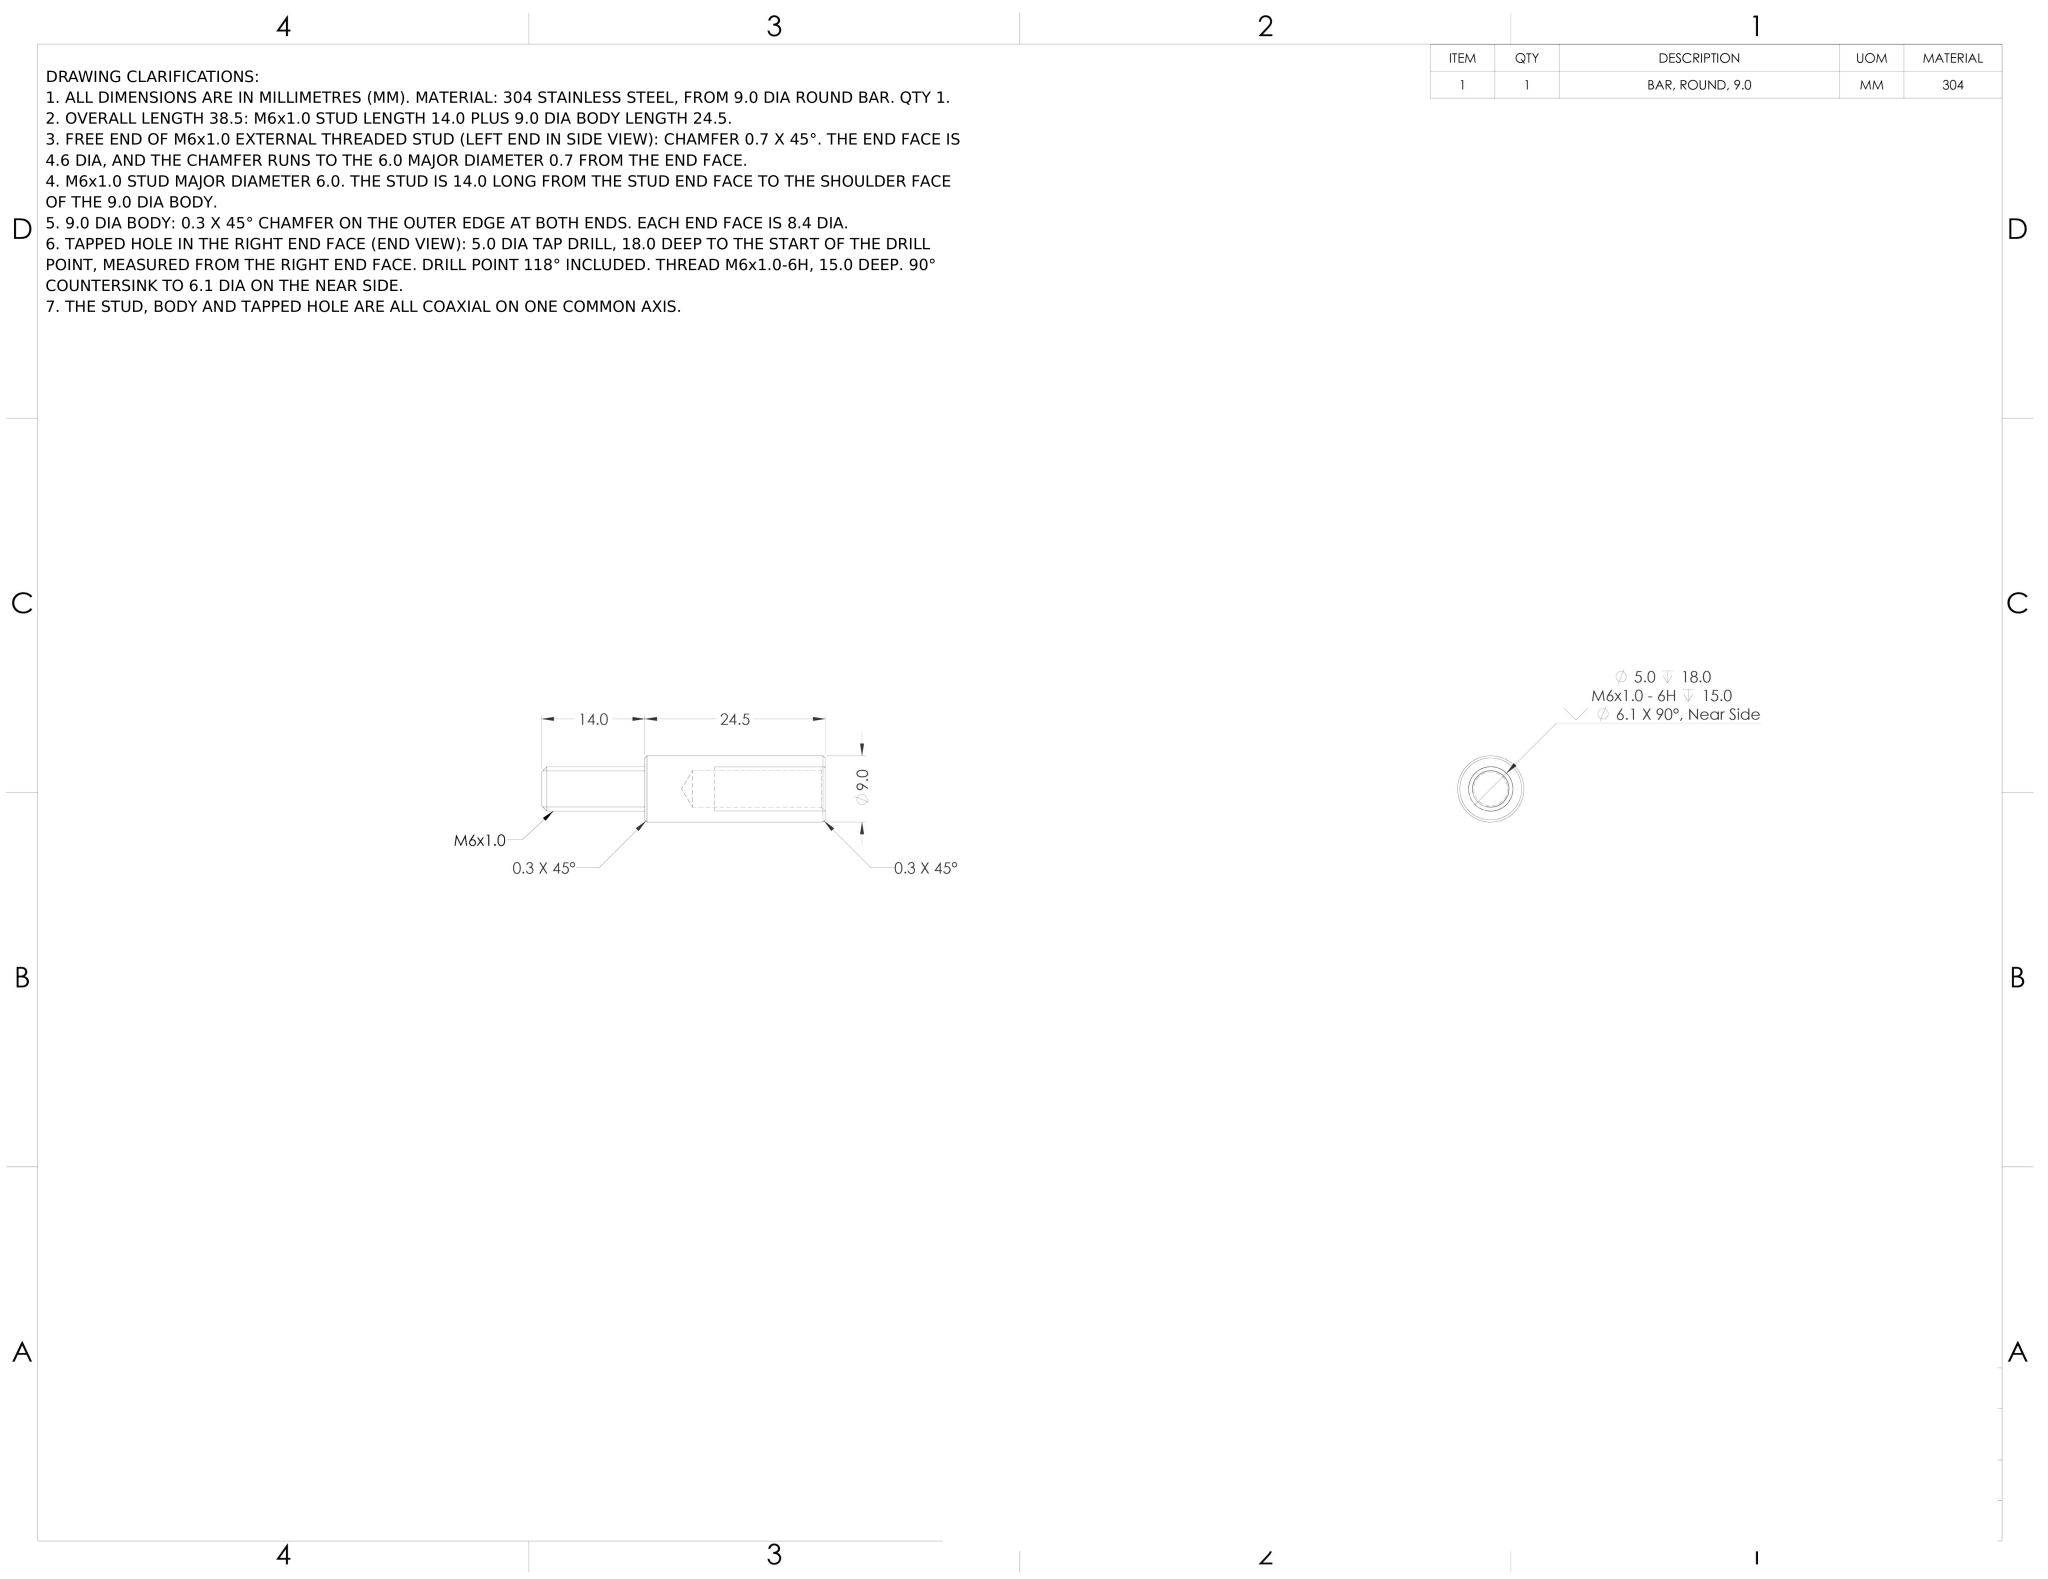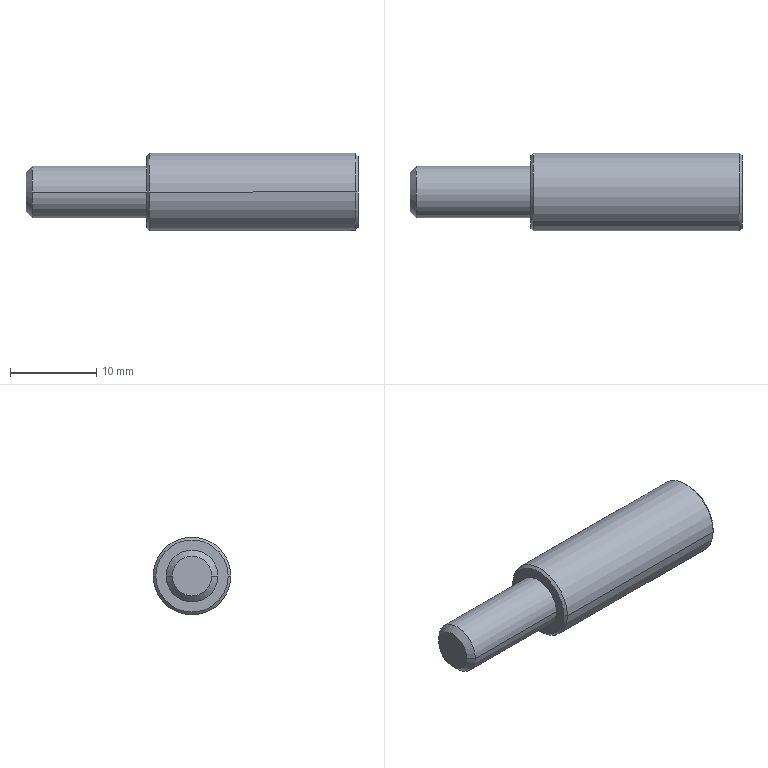Part | NX | mm | Stepped Hollow Cylindrical Connector | 1 solid | 19 faces | box 38.5 x 9 x 9 mm | volume 1582 mm3 | cone 10 | cylinder 6 | plane 3 | commonest cylinder face diameters 5 x2 6 x2 9 x2
STEP:
#1=COLOUR_RGB('',0.9098,0.9176,0.949);
#2=FILL_AREA_STYLE_COLOUR('',#1);
#3=FILL_AREA_STYLE('',(#2));
#4=SURFACE_STYLE_FILL_AREA(#3);
#5=SURFACE_SIDE_STYLE('',(#4));
#6=SURFACE_STYLE_USAGE(.BOTH.,#5);
#7=PRESENTATION_STYLE_ASSIGNMENT((#6));
#8=CARTESIAN_POINT('',(-5.75,0.,2.5));
#9=VERTEX_POINT('',#8);
#10=CARTESIAN_POINT('',(11.725,0.,2.5));
#11=VERTEX_POINT('',#10);
#12=CARTESIAN_POINT('',(12.25,0.,2.5));
#13=DIRECTION('',(1.,0.,0.));
#14=VECTOR('',#13,1000.);
#15=LINE('',#12,#14);
#16=EDGE_CURVE('',#9,#11,#15,.T.);
#17=ORIENTED_EDGE('',*,*,#16,.F.);
#18=CARTESIAN_POINT('',(-5.75,0.,-2.5));
#19=VERTEX_POINT('',#18);
#20=CARTESIAN_POINT('',(-5.75,0.,-0.));
#21=DIRECTION('',(1.,0.,0.));
#22=DIRECTION('',(0.,0.,-1.));
#23=AXIS2_PLACEMENT_3D('',#20,#21,#22);
#24=CIRCLE('',#23,2.5);
#25=EDGE_CURVE('',#19,#9,#24,.T.);
#26=ORIENTED_EDGE('',*,*,#25,.F.);
#27=CARTESIAN_POINT('',(11.725,0.,-2.5));
#28=VERTEX_POINT('',#27);
#29=CARTESIAN_POINT('',(12.25,0.,-2.5));
#30=DIRECTION('',(1.,0.,0.));
#31=VECTOR('',#30,1000.);
#32=LINE('',#29,#31);
#33=EDGE_CURVE('',#19,#28,#32,.T.);
#34=ORIENTED_EDGE('',*,*,#33,.T.);
#35=CARTESIAN_POINT('',(11.725,0.,0.));
#36=DIRECTION('',(1.,0.,0.));
#37=DIRECTION('',(0.,0.,-1.));
#38=AXIS2_PLACEMENT_3D('',#35,#36,#37);
#39=CIRCLE('',#38,2.5);
#40=EDGE_CURVE('',#28,#11,#39,.T.);
#41=ORIENTED_EDGE('',*,*,#40,.T.);
#42=EDGE_LOOP('',(#17,#26,#34,#41));
#43=FACE_OUTER_BOUND('',#42,.T.);
#44=CARTESIAN_POINT('',(12.25,0.,0.));
#45=DIRECTION('',(1.,0.,0.));
#46=DIRECTION('',(0.,0.,-1.));
#47=AXIS2_PLACEMENT_3D('',#44,#45,#46);
#48=CYLINDRICAL_SURFACE('',#47,2.5);
#49=ADVANCED_FACE('',(#43),#48,.F.);
#50=STYLED_ITEM('',(#7),#49);
#51=PRESENTATION_LAYER_ASSIGNMENT('','',(#50));
#52=COLOUR_RGB('',0.9098,0.9176,0.949);
#53=FILL_AREA_STYLE_COLOUR('',#52);
#54=FILL_AREA_STYLE('',(#53));
#55=SURFACE_STYLE_FILL_AREA(#54);
#56=SURFACE_SIDE_STYLE('',(#55));
#57=SURFACE_STYLE_USAGE(.BOTH.,#56);
#58=PRESENTATION_STYLE_ASSIGNMENT((#57));
#59=CARTESIAN_POINT('',(-12.25,3.,-0.));
#60=VERTEX_POINT('',#59);
#61=CARTESIAN_POINT('',(-25.55,3.,-0.));
#62=VERTEX_POINT('',#61);
#63=CARTESIAN_POINT('',(-34.59,3.,-0.));
#64=DIRECTION('',(-1.,-0.,0.));
#65=VECTOR('',#64,1000.);
#66=LINE('',#63,#65);
#67=EDGE_CURVE('',#60,#62,#66,.T.);
#68=ORIENTED_EDGE('',*,*,#67,.F.);
#69=CARTESIAN_POINT('',(-12.25,-3.,-0.));
#70=VERTEX_POINT('',#69);
#71=CARTESIAN_POINT('',(-12.25,0.,-0.));
#72=DIRECTION('',(-1.,-0.,0.));
#73=DIRECTION('',(0.,-1.,0.));
#74=AXIS2_PLACEMENT_3D('',#71,#72,#73);
#75=CIRCLE('',#74,3.);
#76=EDGE_CURVE('',#60,#70,#75,.T.);
#77=ORIENTED_EDGE('',*,*,#76,.T.);
#78=CARTESIAN_POINT('',(-25.55,-3.,-0.));
#79=VERTEX_POINT('',#78);
#80=CARTESIAN_POINT('',(-34.59,-3.,-0.));
#81=DIRECTION('',(-1.,-0.,0.));
#82=VECTOR('',#81,1000.);
#83=LINE('',#80,#82);
#84=EDGE_CURVE('',#70,#79,#83,.T.);
#85=ORIENTED_EDGE('',*,*,#84,.T.);
#86=CARTESIAN_POINT('',(-25.55,0.,-0.));
#87=DIRECTION('',(1.,0.,0.));
#88=DIRECTION('',(0.,1.,0.));
#89=AXIS2_PLACEMENT_3D('',#86,#87,#88);
#90=CIRCLE('',#89,3.);
#91=EDGE_CURVE('',#79,#62,#90,.T.);
#92=ORIENTED_EDGE('',*,*,#91,.T.);
#93=EDGE_LOOP('',(#68,#77,#85,#92));
#94=FACE_OUTER_BOUND('',#93,.T.);
#95=CARTESIAN_POINT('',(-34.59,0.,-0.));
#96=DIRECTION('',(-1.,-0.,0.));
#97=DIRECTION('',(0.,-1.,0.));
#98=AXIS2_PLACEMENT_3D('',#95,#96,#97);
#99=CYLINDRICAL_SURFACE('',#98,3.);
#100=ADVANCED_FACE('',(#94),#99,.T.);
#101=STYLED_ITEM('',(#58),#100);
#102=(LENGTH_UNIT()NAMED_UNIT(*)SI_UNIT(.MILLI.,.METRE.));
#103=UNCERTAINTY_MEASURE_WITH_UNIT(LENGTH_MEASURE(0.00001),#102,'','');
#104=(NAMED_UNIT(*)PLANE_ANGLE_UNIT()SI_UNIT($,.RADIAN.));
#105=(NAMED_UNIT(*)SI_UNIT($,.STERADIAN.)SOLID_ANGLE_UNIT());
#106=(GEOMETRIC_REPRESENTATION_CONTEXT(3)GLOBAL_UNCERTAINTY_ASSIGNED_CONTEXT((#103))GLOBAL_UNIT_ASSIGNED_CONTEXT((#102,#104,#105))REPRESENTATION_CONTEXT('',''));
#107=MECHANICAL_DESIGN_GEOMETRIC_PRESENTATION_REPRESENTATION('',(#101),#106);
#108=COLOUR_RGB('',0.9098,0.9176,0.949);
#109=FILL_AREA_STYLE_COLOUR('',#108);
#110=FILL_AREA_STYLE('',(#109));
#111=SURFACE_STYLE_FILL_AREA(#110);
#112=SURFACE_SIDE_STYLE('',(#111));
#113=SURFACE_STYLE_USAGE(.BOTH.,#112);
#114=PRESENTATION_STYLE_ASSIGNMENT((#113));
#115=CARTESIAN_POINT('',(-12.25,-4.2,-0.));
#116=VERTEX_POINT('',#115);
#117=CARTESIAN_POINT('',(-12.25,4.2,-0.));
#118=VERTEX_POINT('',#117);
#119=CARTESIAN_POINT('',(-12.25,0.,-0.));
#120=DIRECTION('',(-1.,-0.,0.));
#121=DIRECTION('',(0.,1.,0.));
#122=AXIS2_PLACEMENT_3D('',#119,#120,#121);
#123=CIRCLE('',#122,4.2);
#124=EDGE_CURVE('',#116,#118,#123,.T.);
#125=ORIENTED_EDGE('',*,*,#124,.F.);
#126=CARTESIAN_POINT('',(-11.95,-4.5,-0.));
#127=VERTEX_POINT('',#126);
#128=CARTESIAN_POINT('',(-12.25,-4.2,-0.));
#129=DIRECTION('',(0.7071,-0.7071,0.));
#130=VECTOR('',#129,1000.);
#131=LINE('',#128,#130);
#132=EDGE_CURVE('',#116,#127,#131,.T.);
#133=ORIENTED_EDGE('',*,*,#132,.T.);
#134=CARTESIAN_POINT('',(-11.95,4.5,-0.));
#135=VERTEX_POINT('',#134);
#136=CARTESIAN_POINT('',(-11.95,0.,-0.));
#137=DIRECTION('',(1.,0.,0.));
#138=DIRECTION('',(0.,1.,0.));
#139=AXIS2_PLACEMENT_3D('',#136,#137,#138);
#140=CIRCLE('',#139,4.5);
#141=EDGE_CURVE('',#135,#127,#140,.T.);
#142=ORIENTED_EDGE('',*,*,#141,.F.);
#143=CARTESIAN_POINT('',(-12.25,4.2,-0.));
#144=DIRECTION('',(0.7071,0.7071,0.));
#145=VECTOR('',#144,1000.);
#146=LINE('',#143,#145);
#147=EDGE_CURVE('',#118,#135,#146,.T.);
#148=ORIENTED_EDGE('',*,*,#147,.F.);
#149=EDGE_LOOP('',(#125,#133,#142,#148));
#150=FACE_OUTER_BOUND('',#149,.T.);
#151=CARTESIAN_POINT('',(-12.25,0.,-0.));
#152=DIRECTION('',(1.,0.,0.));
#153=DIRECTION('',(0.,1.,0.));
#154=AXIS2_PLACEMENT_3D('',#151,#152,#153);
#155=CONICAL_SURFACE('',#154,4.2,0.7854);
#156=ADVANCED_FACE('',(#150),#155,.T.);
#157=CARTESIAN_POINT('',(12.25,4.2,0.));
#158=VERTEX_POINT('',#157);
#159=CARTESIAN_POINT('',(12.25,-4.2,0.));
#160=VERTEX_POINT('',#159);
#161=CARTESIAN_POINT('',(12.25,0.,0.));
#162=DIRECTION('',(1.,0.,0.));
#163=DIRECTION('',(0.,-1.,0.));
#164=AXIS2_PLACEMENT_3D('',#161,#162,#163);
#165=CIRCLE('',#164,4.2);
#166=EDGE_CURVE('',#158,#160,#165,.T.);
#167=ORIENTED_EDGE('',*,*,#166,.F.);
#168=CARTESIAN_POINT('',(11.95,4.5,-0.));
#169=VERTEX_POINT('',#168);
#170=CARTESIAN_POINT('',(11.95,4.5,0.));
#171=DIRECTION('',(-0.7071,0.7071,0.));
#172=VECTOR('',#171,1000.);
#173=LINE('',#170,#172);
#174=EDGE_CURVE('',#158,#169,#173,.T.);
#175=ORIENTED_EDGE('',*,*,#174,.T.);
#176=CARTESIAN_POINT('',(11.95,-4.5,0.));
#177=VERTEX_POINT('',#176);
#178=CARTESIAN_POINT('',(11.95,0.,0.));
#179=DIRECTION('',(-1.,-0.,0.));
#180=DIRECTION('',(0.,-1.,0.));
#181=AXIS2_PLACEMENT_3D('',#178,#179,#180);
#182=CIRCLE('',#181,4.5);
#183=EDGE_CURVE('',#177,#169,#182,.T.);
#184=ORIENTED_EDGE('',*,*,#183,.F.);
#185=CARTESIAN_POINT('',(11.95,-4.5,0.));
#186=DIRECTION('',(-0.7071,-0.7071,0.));
#187=VECTOR('',#186,1000.);
#188=LINE('',#185,#187);
#189=EDGE_CURVE('',#160,#177,#188,.T.);
#190=ORIENTED_EDGE('',*,*,#189,.F.);
#191=EDGE_LOOP('',(#167,#175,#184,#190));
#192=FACE_OUTER_BOUND('',#191,.T.);
#193=CARTESIAN_POINT('',(11.95,0.,0.));
#194=DIRECTION('',(-1.,-0.,0.));
#195=DIRECTION('',(0.,-1.,0.));
#196=AXIS2_PLACEMENT_3D('',#193,#194,#195);
#197=CONICAL_SURFACE('',#196,4.5,0.7854);
#198=ADVANCED_FACE('',(#192),#197,.T.);
#199=CARTESIAN_POINT('',(-26.25,-2.3,-0.));
#200=VERTEX_POINT('',#199);
#201=CARTESIAN_POINT('',(-26.25,2.3,-0.));
#202=VERTEX_POINT('',#201);
#203=CARTESIAN_POINT('',(-26.25,0.,-0.));
#204=DIRECTION('',(-1.,-0.,0.));
#205=DIRECTION('',(0.,1.,0.));
#206=AXIS2_PLACEMENT_3D('',#203,#204,#205);
#207=CIRCLE('',#206,2.3);
#208=EDGE_CURVE('',#200,#202,#207,.T.);
#209=ORIENTED_EDGE('',*,*,#208,.F.);
#210=CARTESIAN_POINT('',(-26.25,-2.3,-0.));
#211=DIRECTION('',(0.7071,-0.7071,0.));
#212=VECTOR('',#211,1000.);
#213=LINE('',#210,#212);
#214=EDGE_CURVE('',#200,#79,#213,.T.);
#215=ORIENTED_EDGE('',*,*,#214,.T.);
#216=CARTESIAN_POINT('',(-25.55,0.,-0.));
#217=DIRECTION('',(1.,0.,0.));
#218=DIRECTION('',(0.,1.,0.));
#219=AXIS2_PLACEMENT_3D('',#216,#217,#218);
#220=CIRCLE('',#219,3.);
#221=EDGE_CURVE('',#62,#79,#220,.T.);
#222=ORIENTED_EDGE('',*,*,#221,.F.);
#223=CARTESIAN_POINT('',(-26.25,2.3,-0.));
#224=DIRECTION('',(0.7071,0.7071,0.));
#225=VECTOR('',#224,1000.);
#226=LINE('',#223,#225);
#227=EDGE_CURVE('',#202,#62,#226,.T.);
#228=ORIENTED_EDGE('',*,*,#227,.F.);
#229=EDGE_LOOP('',(#209,#215,#222,#228));
#230=FACE_OUTER_BOUND('',#229,.T.);
#231=CARTESIAN_POINT('',(-26.25,0.,-0.));
#232=DIRECTION('',(1.,0.,0.));
#233=DIRECTION('',(0.,1.,0.));
#234=AXIS2_PLACEMENT_3D('',#231,#232,#233);
#235=CONICAL_SURFACE('',#234,2.3,0.7854);
#236=ADVANCED_FACE('',(#230),#235,.T.);
#237=CARTESIAN_POINT('',(11.725,0.,0.));
#238=DIRECTION('',(1.,0.,0.));
#239=DIRECTION('',(0.,0.,-1.));
#240=AXIS2_PLACEMENT_3D('',#237,#238,#239);
#241=CIRCLE('',#240,2.5);
#242=EDGE_CURVE('',#11,#28,#241,.T.);
#243=ORIENTED_EDGE('',*,*,#242,.F.);
#244=CARTESIAN_POINT('',(12.25,0.,3.025));
#245=VERTEX_POINT('',#244);
#246=CARTESIAN_POINT('',(12.25,0.,3.025));
#247=DIRECTION('',(0.7071,0.,0.7071));
#248=VECTOR('',#247,1000.);
#249=LINE('',#246,#248);
#250=EDGE_CURVE('',#11,#245,#249,.T.);
#251=ORIENTED_EDGE('',*,*,#250,.T.);
#252=CARTESIAN_POINT('',(12.25,0.,-3.025));
#253=VERTEX_POINT('',#252);
#254=CARTESIAN_POINT('',(12.25,0.,0.));
#255=DIRECTION('',(1.,0.,0.));
#256=DIRECTION('',(0.,0.,-1.));
#257=AXIS2_PLACEMENT_3D('',#254,#255,#256);
#258=CIRCLE('',#257,3.025);
#259=EDGE_CURVE('',#245,#253,#258,.T.);
#260=ORIENTED_EDGE('',*,*,#259,.T.);
#261=CARTESIAN_POINT('',(12.25,0.,-3.025));
#262=DIRECTION('',(0.7071,0.,-0.7071));
#263=VECTOR('',#262,1000.);
#264=LINE('',#261,#263);
#265=EDGE_CURVE('',#28,#253,#264,.T.);
#266=ORIENTED_EDGE('',*,*,#265,.F.);
#267=EDGE_LOOP('',(#243,#251,#260,#266));
#268=FACE_OUTER_BOUND('',#267,.T.);
#269=CARTESIAN_POINT('',(12.25,0.,0.));
#270=DIRECTION('',(1.,0.,0.));
#271=DIRECTION('',(0.,0.,-1.));
#272=AXIS2_PLACEMENT_3D('',#269,#270,#271);
#273=CONICAL_SURFACE('',#272,3.025,0.7854);
#274=ADVANCED_FACE('',(#268),#273,.F.);
#275=CARTESIAN_POINT('',(-5.75,0.,-0.));
#276=DIRECTION('',(1.,0.,0.));
#277=DIRECTION('',(0.,0.,-1.));
#278=AXIS2_PLACEMENT_3D('',#275,#276,#277);
#279=CIRCLE('',#278,2.5);
#280=EDGE_CURVE('',#9,#19,#279,.T.);
#281=ORIENTED_EDGE('',*,*,#280,.F.);
#282=ORIENTED_EDGE('',*,*,#16,.T.);
#283=ORIENTED_EDGE('',*,*,#242,.T.);
#284=ORIENTED_EDGE('',*,*,#33,.F.);
#285=EDGE_LOOP('',(#281,#282,#283,#284));
#286=FACE_OUTER_BOUND('',#285,.T.);
#287=CARTESIAN_POINT('',(12.25,0.,0.));
#288=DIRECTION('',(1.,0.,0.));
#289=DIRECTION('',(0.,0.,-1.));
#290=AXIS2_PLACEMENT_3D('',#287,#288,#289);
#291=CYLINDRICAL_SURFACE('',#290,2.5);
#292=ADVANCED_FACE('',(#286),#291,.F.);
#293=CARTESIAN_POINT('',(-7.252,0.,-0.));
#294=VERTEX_POINT('',#293);
#295=CARTESIAN_POINT('',(-5.75,0.,-2.5));
#296=DIRECTION('',(0.515,0.,-0.8572));
#297=VECTOR('',#296,1000.);
#298=LINE('',#295,#297);
#299=EDGE_CURVE('',#294,#19,#298,.T.);
#300=ORIENTED_EDGE('',*,*,#299,.F.);
#301=CARTESIAN_POINT('',(-5.75,0.,2.5));
#302=DIRECTION('',(0.515,0.,0.8572));
#303=VECTOR('',#302,1000.);
#304=LINE('',#301,#303);
#305=EDGE_CURVE('',#294,#9,#304,.T.);
#306=ORIENTED_EDGE('',*,*,#305,.T.);
#307=ORIENTED_EDGE('',*,*,#280,.T.);
#308=EDGE_LOOP('',(#300,#306,#307));
#309=FACE_OUTER_BOUND('',#308,.T.);
#310=CARTESIAN_POINT('',(-5.75,0.,-0.));
#311=DIRECTION('',(1.,0.,0.));
#312=DIRECTION('',(0.,0.,-1.));
#313=AXIS2_PLACEMENT_3D('',#310,#311,#312);
#314=CONICAL_SURFACE('',#313,2.5,1.03);
#315=ADVANCED_FACE('',(#309),#314,.F.);
#316=CARTESIAN_POINT('',(-12.25,0.,-0.));
#317=DIRECTION('',(-1.,-0.,0.));
#318=DIRECTION('',(0.,-1.,0.));
#319=AXIS2_PLACEMENT_3D('',#316,#317,#318);
#320=CIRCLE('',#319,3.);
#321=EDGE_CURVE('',#70,#60,#320,.T.);
#322=ORIENTED_EDGE('',*,*,#321,.T.);
#323=ORIENTED_EDGE('',*,*,#67,.T.);
#324=ORIENTED_EDGE('',*,*,#221,.T.);
#325=ORIENTED_EDGE('',*,*,#84,.F.);
#326=EDGE_LOOP('',(#322,#323,#324,#325));
#327=FACE_OUTER_BOUND('',#326,.T.);
#328=CARTESIAN_POINT('',(-34.59,0.,-0.));
#329=DIRECTION('',(-1.,-0.,0.));
#330=DIRECTION('',(0.,-1.,0.));
#331=AXIS2_PLACEMENT_3D('',#328,#329,#330);
#332=CYLINDRICAL_SURFACE('',#331,3.);
#333=ADVANCED_FACE('',(#327),#332,.T.);
#334=ORIENTED_EDGE('',*,*,#183,.T.);
#335=CARTESIAN_POINT('',(-34.59,4.5,-0.));
#336=DIRECTION('',(-1.,-0.,0.));
#337=VECTOR('',#336,1000.);
#338=LINE('',#335,#337);
#339=EDGE_CURVE('',#169,#135,#338,.T.);
#340=ORIENTED_EDGE('',*,*,#339,.T.);
#341=ORIENTED_EDGE('',*,*,#141,.T.);
#342=CARTESIAN_POINT('',(-34.59,-4.5,-0.));
#343=DIRECTION('',(-1.,-0.,0.));
#344=VECTOR('',#343,1000.);
#345=LINE('',#342,#344);
#346=EDGE_CURVE('',#177,#127,#345,.T.);
#347=ORIENTED_EDGE('',*,*,#346,.F.);
#348=EDGE_LOOP('',(#334,#340,#341,#347));
#349=FACE_OUTER_BOUND('',#348,.T.);
#350=CARTESIAN_POINT('',(-34.59,0.,-0.));
#351=DIRECTION('',(-1.,-0.,0.));
#352=DIRECTION('',(0.,-1.,0.));
#353=AXIS2_PLACEMENT_3D('',#350,#351,#352);
#354=CYLINDRICAL_SURFACE('',#353,4.5);
#355=ADVANCED_FACE('',(#349),#354,.T.);
#356=CARTESIAN_POINT('',(-26.25,0.,-0.));
#357=DIRECTION('',(-1.,-0.,0.));
#358=DIRECTION('',(0.,1.,0.));
#359=AXIS2_PLACEMENT_3D('',#356,#357,#358);
#360=CIRCLE('',#359,2.3);
#361=EDGE_CURVE('',#202,#200,#360,.T.);
#362=ORIENTED_EDGE('',*,*,#361,.T.);
#363=ORIENTED_EDGE('',*,*,#208,.T.);
#364=EDGE_LOOP('',(#362,#363));
#365=FACE_OUTER_BOUND('',#364,.T.);
#366=CARTESIAN_POINT('',(-26.25,3.,-0.));
#367=DIRECTION('',(1.,0.,0.));
#368=DIRECTION('',(-0.,1.,0.));
#369=AXIS2_PLACEMENT_3D('',#366,#367,#368);
#370=PLANE('',#369);
#371=ADVANCED_FACE('',(#365),#370,.F.);
#372=CARTESIAN_POINT('',(12.25,0.,0.));
#373=DIRECTION('',(1.,0.,0.));
#374=DIRECTION('',(0.,-1.,0.));
#375=AXIS2_PLACEMENT_3D('',#372,#373,#374);
#376=CIRCLE('',#375,4.2);
#377=EDGE_CURVE('',#160,#158,#376,.T.);
#378=ORIENTED_EDGE('',*,*,#377,.T.);
#379=ORIENTED_EDGE('',*,*,#166,.T.);
#380=EDGE_LOOP('',(#378,#379));
#381=FACE_OUTER_BOUND('',#380,.T.);
#382=CARTESIAN_POINT('',(12.25,0.,0.));
#383=DIRECTION('',(1.,0.,0.));
#384=DIRECTION('',(0.,0.,-1.));
#385=AXIS2_PLACEMENT_3D('',#382,#383,#384);
#386=CIRCLE('',#385,3.025);
#387=EDGE_CURVE('',#253,#245,#386,.T.);
#388=ORIENTED_EDGE('',*,*,#387,.F.);
#389=ORIENTED_EDGE('',*,*,#259,.F.);
#390=EDGE_LOOP('',(#388,#389));
#391=FACE_BOUND('',#390,.T.);
#392=CARTESIAN_POINT('',(12.25,0.,0.));
#393=DIRECTION('',(-1.,-0.,0.));
#394=DIRECTION('',(0.,-1.,0.));
#395=AXIS2_PLACEMENT_3D('',#392,#393,#394);
#396=PLANE('',#395);
#397=ADVANCED_FACE('',(#381,#391),#396,.F.);
#398=ORIENTED_EDGE('',*,*,#339,.F.);
#399=CARTESIAN_POINT('',(11.95,0.,0.));
#400=DIRECTION('',(-1.,-0.,0.));
#401=DIRECTION('',(0.,-1.,0.));
#402=AXIS2_PLACEMENT_3D('',#399,#400,#401);
#403=CIRCLE('',#402,4.5);
#404=EDGE_CURVE('',#169,#177,#403,.T.);
#405=ORIENTED_EDGE('',*,*,#404,.T.);
#406=ORIENTED_EDGE('',*,*,#346,.T.);
#407=CARTESIAN_POINT('',(-11.95,0.,-0.));
#408=DIRECTION('',(1.,0.,0.));
#409=DIRECTION('',(0.,1.,0.));
#410=AXIS2_PLACEMENT_3D('',#407,#408,#409);
#411=CIRCLE('',#410,4.5);
#412=EDGE_CURVE('',#127,#135,#411,.T.);
#413=ORIENTED_EDGE('',*,*,#412,.T.);
#414=EDGE_LOOP('',(#398,#405,#406,#413));
#415=FACE_OUTER_BOUND('',#414,.T.);
#416=CARTESIAN_POINT('',(-34.59,0.,-0.));
#417=DIRECTION('',(-1.,-0.,0.));
#418=DIRECTION('',(0.,-1.,0.));
#419=AXIS2_PLACEMENT_3D('',#416,#417,#418);
#420=CYLINDRICAL_SURFACE('',#419,4.5);
#421=ADVANCED_FACE('',(#415),#420,.T.);
#422=CARTESIAN_POINT('',(-12.25,0.,-0.));
#423=DIRECTION('',(-1.,-0.,0.));
#424=DIRECTION('',(0.,1.,0.));
#425=AXIS2_PLACEMENT_3D('',#422,#423,#424);
#426=CIRCLE('',#425,4.2);
#427=EDGE_CURVE('',#118,#116,#426,.T.);
#428=ORIENTED_EDGE('',*,*,#427,.T.);
#429=ORIENTED_EDGE('',*,*,#124,.T.);
#430=EDGE_LOOP('',(#428,#429));
#431=FACE_OUTER_BOUND('',#430,.T.);
#432=ORIENTED_EDGE('',*,*,#321,.F.);
#433=ORIENTED_EDGE('',*,*,#76,.F.);
#434=EDGE_LOOP('',(#432,#433));
#435=FACE_BOUND('',#434,.T.);
#436=CARTESIAN_POINT('',(-12.25,4.5,-0.));
#437=DIRECTION('',(1.,0.,0.));
#438=DIRECTION('',(-0.,1.,0.));
#439=AXIS2_PLACEMENT_3D('',#436,#437,#438);
#440=PLANE('',#439);
#441=ADVANCED_FACE('',(#431,#435),#440,.F.);
#442=ORIENTED_EDGE('',*,*,#305,.F.);
#443=ORIENTED_EDGE('',*,*,#299,.T.);
#444=ORIENTED_EDGE('',*,*,#25,.T.);
#445=EDGE_LOOP('',(#442,#443,#444));
#446=FACE_OUTER_BOUND('',#445,.T.);
#447=CARTESIAN_POINT('',(-5.75,0.,-0.));
#448=DIRECTION('',(1.,0.,0.));
#449=DIRECTION('',(0.,0.,-1.));
#450=AXIS2_PLACEMENT_3D('',#447,#448,#449);
#451=CONICAL_SURFACE('',#450,2.5,1.03);
#452=ADVANCED_FACE('',(#446),#451,.F.);
#453=ORIENTED_EDGE('',*,*,#250,.F.);
#454=ORIENTED_EDGE('',*,*,#40,.F.);
#455=ORIENTED_EDGE('',*,*,#265,.T.);
#456=ORIENTED_EDGE('',*,*,#387,.T.);
#457=EDGE_LOOP('',(#453,#454,#455,#456));
#458=FACE_OUTER_BOUND('',#457,.T.);
#459=CARTESIAN_POINT('',(12.25,0.,0.));
#460=DIRECTION('',(1.,0.,0.));
#461=DIRECTION('',(0.,0.,-1.));
#462=AXIS2_PLACEMENT_3D('',#459,#460,#461);
#463=CONICAL_SURFACE('',#462,3.025,0.7854);
#464=ADVANCED_FACE('',(#458),#463,.F.);
#465=ORIENTED_EDGE('',*,*,#214,.F.);
#466=ORIENTED_EDGE('',*,*,#361,.F.);
#467=ORIENTED_EDGE('',*,*,#227,.T.);
#468=ORIENTED_EDGE('',*,*,#91,.F.);
#469=EDGE_LOOP('',(#465,#466,#467,#468));
#470=FACE_OUTER_BOUND('',#469,.T.);
#471=CARTESIAN_POINT('',(-26.25,0.,-0.));
#472=DIRECTION('',(1.,0.,0.));
#473=DIRECTION('',(0.,1.,0.));
#474=AXIS2_PLACEMENT_3D('',#471,#472,#473);
#475=CONICAL_SURFACE('',#474,2.3,0.7854);
#476=ADVANCED_FACE('',(#470),#475,.T.);
#477=ORIENTED_EDGE('',*,*,#174,.F.);
#478=ORIENTED_EDGE('',*,*,#377,.F.);
#479=ORIENTED_EDGE('',*,*,#189,.T.);
#480=ORIENTED_EDGE('',*,*,#404,.F.);
#481=EDGE_LOOP('',(#477,#478,#479,#480));
#482=FACE_OUTER_BOUND('',#481,.T.);
#483=CARTESIAN_POINT('',(11.95,0.,0.));
#484=DIRECTION('',(-1.,-0.,0.));
#485=DIRECTION('',(0.,-1.,0.));
#486=AXIS2_PLACEMENT_3D('',#483,#484,#485);
#487=CONICAL_SURFACE('',#486,4.5,0.7854);
#488=ADVANCED_FACE('',(#482),#487,.T.);
#489=ORIENTED_EDGE('',*,*,#132,.F.);
#490=ORIENTED_EDGE('',*,*,#427,.F.);
#491=ORIENTED_EDGE('',*,*,#147,.T.);
#492=ORIENTED_EDGE('',*,*,#412,.F.);
#493=EDGE_LOOP('',(#489,#490,#491,#492));
#494=FACE_OUTER_BOUND('',#493,.T.);
#495=CARTESIAN_POINT('',(-12.25,0.,-0.));
#496=DIRECTION('',(1.,0.,0.));
#497=DIRECTION('',(0.,1.,0.));
#498=AXIS2_PLACEMENT_3D('',#495,#496,#497);
#499=CONICAL_SURFACE('',#498,4.2,0.7854);
#500=ADVANCED_FACE('',(#494),#499,.T.);
#501=CLOSED_SHELL('',(#156,#198,#236,#274,#292,#315,#333,#355,#371,#397,#421,#441,#100,#452,#49,#464,#476,#488,#500));
#502=MANIFOLD_SOLID_BREP('',#501);
#503=STYLED_ITEM('',(#114),#502);
#504=(LENGTH_UNIT()NAMED_UNIT(*)SI_UNIT(.MILLI.,.METRE.));
#505=UNCERTAINTY_MEASURE_WITH_UNIT(LENGTH_MEASURE(0.00001),#504,'','');
#506=(NAMED_UNIT(*)PLANE_ANGLE_UNIT()SI_UNIT($,.RADIAN.));
#507=(NAMED_UNIT(*)SI_UNIT($,.STERADIAN.)SOLID_ANGLE_UNIT());
#508=(GEOMETRIC_REPRESENTATION_CONTEXT(3)GLOBAL_UNCERTAINTY_ASSIGNED_CONTEXT((#505))GLOBAL_UNIT_ASSIGNED_CONTEXT((#504,#506,#507))REPRESENTATION_CONTEXT('',''));
#509=MECHANICAL_DESIGN_GEOMETRIC_PRESENTATION_REPRESENTATION('',(#503),#508);
#510=COLOUR_RGB('',0.9098,0.9176,0.949);
#511=FILL_AREA_STYLE_COLOUR('',#510);
#512=FILL_AREA_STYLE('',(#511));
#513=SURFACE_STYLE_FILL_AREA(#512);
#514=SURFACE_SIDE_STYLE('',(#513));
#515=SURFACE_STYLE_USAGE(.BOTH.,#514);
#516=PRESENTATION_STYLE_ASSIGNMENT((#515));
#517=CARTESIAN_POINT('',(0.,0.,0.));
#518=DIRECTION('',(0.,0.,1.));
#519=DIRECTION('',(1.,0.,0.));
#520=AXIS2_PLACEMENT_3D('',#517,#518,#519);
#521=(LENGTH_UNIT()NAMED_UNIT(*)SI_UNIT(.MILLI.,.METRE.));
#522=UNCERTAINTY_MEASURE_WITH_UNIT(LENGTH_MEASURE(0.00001),#521,'','');
#523=(NAMED_UNIT(*)PLANE_ANGLE_UNIT()SI_UNIT($,.RADIAN.));
#524=(NAMED_UNIT(*)SI_UNIT($,.STERADIAN.)SOLID_ANGLE_UNIT());
#525=(GEOMETRIC_REPRESENTATION_CONTEXT(3)GLOBAL_UNCERTAINTY_ASSIGNED_CONTEXT((#522))GLOBAL_UNIT_ASSIGNED_CONTEXT((#521,#523,#524))REPRESENTATION_CONTEXT('',''));
#526=ADVANCED_BREP_SHAPE_REPRESENTATION('',(#502,#520),#525);
#527=STYLED_ITEM('',(#516),#526);
#528=PRESENTATION_LAYER_ASSIGNMENT('','',(#527));
#529=COLOUR_RGB('',0.9098,0.9176,0.949);
#530=FILL_AREA_STYLE_COLOUR('',#529);
#531=FILL_AREA_STYLE('',(#530));
#532=SURFACE_STYLE_FILL_AREA(#531);
#533=SURFACE_SIDE_STYLE('',(#532));
#534=SURFACE_STYLE_USAGE(.BOTH.,#533);
#535=PRESENTATION_STYLE_ASSIGNMENT((#534));
#536=STYLED_ITEM('',(#535),#292);
#537=PRESENTATION_LAYER_ASSIGNMENT('','',(#536));
#538=COLOUR_RGB('',0.9098,0.9176,0.949);
#539=FILL_AREA_STYLE_COLOUR('',#538);
#540=FILL_AREA_STYLE('',(#539));
#541=SURFACE_STYLE_FILL_AREA(#540);
#542=SURFACE_SIDE_STYLE('',(#541));
#543=SURFACE_STYLE_USAGE(.BOTH.,#542);
#544=PRESENTATION_STYLE_ASSIGNMENT((#543));
#545=STYLED_ITEM('',(#544),#333);
#546=PRESENTATION_LAYER_ASSIGNMENT('','',(#545));
#547=PRESENTATION_LAYER_ASSIGNMENT('','',(#503));
#548=(LENGTH_UNIT()NAMED_UNIT(*)SI_UNIT(.MILLI.,.METRE.));
#549=UNCERTAINTY_MEASURE_WITH_UNIT(LENGTH_MEASURE(0.00001),#548,'','');
#550=(NAMED_UNIT(*)PLANE_ANGLE_UNIT()SI_UNIT($,.RADIAN.));
#551=(NAMED_UNIT(*)SI_UNIT($,.STERADIAN.)SOLID_ANGLE_UNIT());
#552=(GEOMETRIC_REPRESENTATION_CONTEXT(3)GLOBAL_UNCERTAINTY_ASSIGNED_CONTEXT((#549))GLOBAL_UNIT_ASSIGNED_CONTEXT((#548,#550,#551))REPRESENTATION_CONTEXT('',''));
#553=MECHANICAL_DESIGN_GEOMETRIC_PRESENTATION_REPRESENTATION('',(#545),#552);
#554=(LENGTH_UNIT()NAMED_UNIT(*)SI_UNIT(.MILLI.,.METRE.));
#555=UNCERTAINTY_MEASURE_WITH_UNIT(LENGTH_MEASURE(0.00001),#554,'','');
#556=(NAMED_UNIT(*)PLANE_ANGLE_UNIT()SI_UNIT($,.RADIAN.));
#557=(NAMED_UNIT(*)SI_UNIT($,.STERADIAN.)SOLID_ANGLE_UNIT());
#558=(GEOMETRIC_REPRESENTATION_CONTEXT(3)GLOBAL_UNCERTAINTY_ASSIGNED_CONTEXT((#555))GLOBAL_UNIT_ASSIGNED_CONTEXT((#554,#556,#557))REPRESENTATION_CONTEXT('',''));
#559=MECHANICAL_DESIGN_GEOMETRIC_PRESENTATION_REPRESENTATION('',(#50),#558);
#560=(LENGTH_UNIT()NAMED_UNIT(*)SI_UNIT(.MILLI.,.METRE.));
#561=UNCERTAINTY_MEASURE_WITH_UNIT(LENGTH_MEASURE(0.00001),#560,'','');
#562=(NAMED_UNIT(*)PLANE_ANGLE_UNIT()SI_UNIT($,.RADIAN.));
#563=(NAMED_UNIT(*)SI_UNIT($,.STERADIAN.)SOLID_ANGLE_UNIT());
#564=(GEOMETRIC_REPRESENTATION_CONTEXT(3)GLOBAL_UNCERTAINTY_ASSIGNED_CONTEXT((#561))GLOBAL_UNIT_ASSIGNED_CONTEXT((#560,#562,#563))REPRESENTATION_CONTEXT('',''));
#565=MECHANICAL_DESIGN_GEOMETRIC_PRESENTATION_REPRESENTATION('',(#536),#564);
#566=(LENGTH_UNIT()NAMED_UNIT(*)SI_UNIT(.MILLI.,.METRE.));
#567=UNCERTAINTY_MEASURE_WITH_UNIT(LENGTH_MEASURE(0.00001),#566,'','');
#568=(NAMED_UNIT(*)PLANE_ANGLE_UNIT()SI_UNIT($,.RADIAN.));
#569=(NAMED_UNIT(*)SI_UNIT($,.STERADIAN.)SOLID_ANGLE_UNIT());
#570=(GEOMETRIC_REPRESENTATION_CONTEXT(3)GLOBAL_UNCERTAINTY_ASSIGNED_CONTEXT((#567))GLOBAL_UNIT_ASSIGNED_CONTEXT((#566,#568,#569))REPRESENTATION_CONTEXT('',''));
#571=MECHANICAL_DESIGN_GEOMETRIC_PRESENTATION_REPRESENTATION('',(#527),#570);
#572=PRESENTATION_LAYER_ASSIGNMENT('','',(#101));